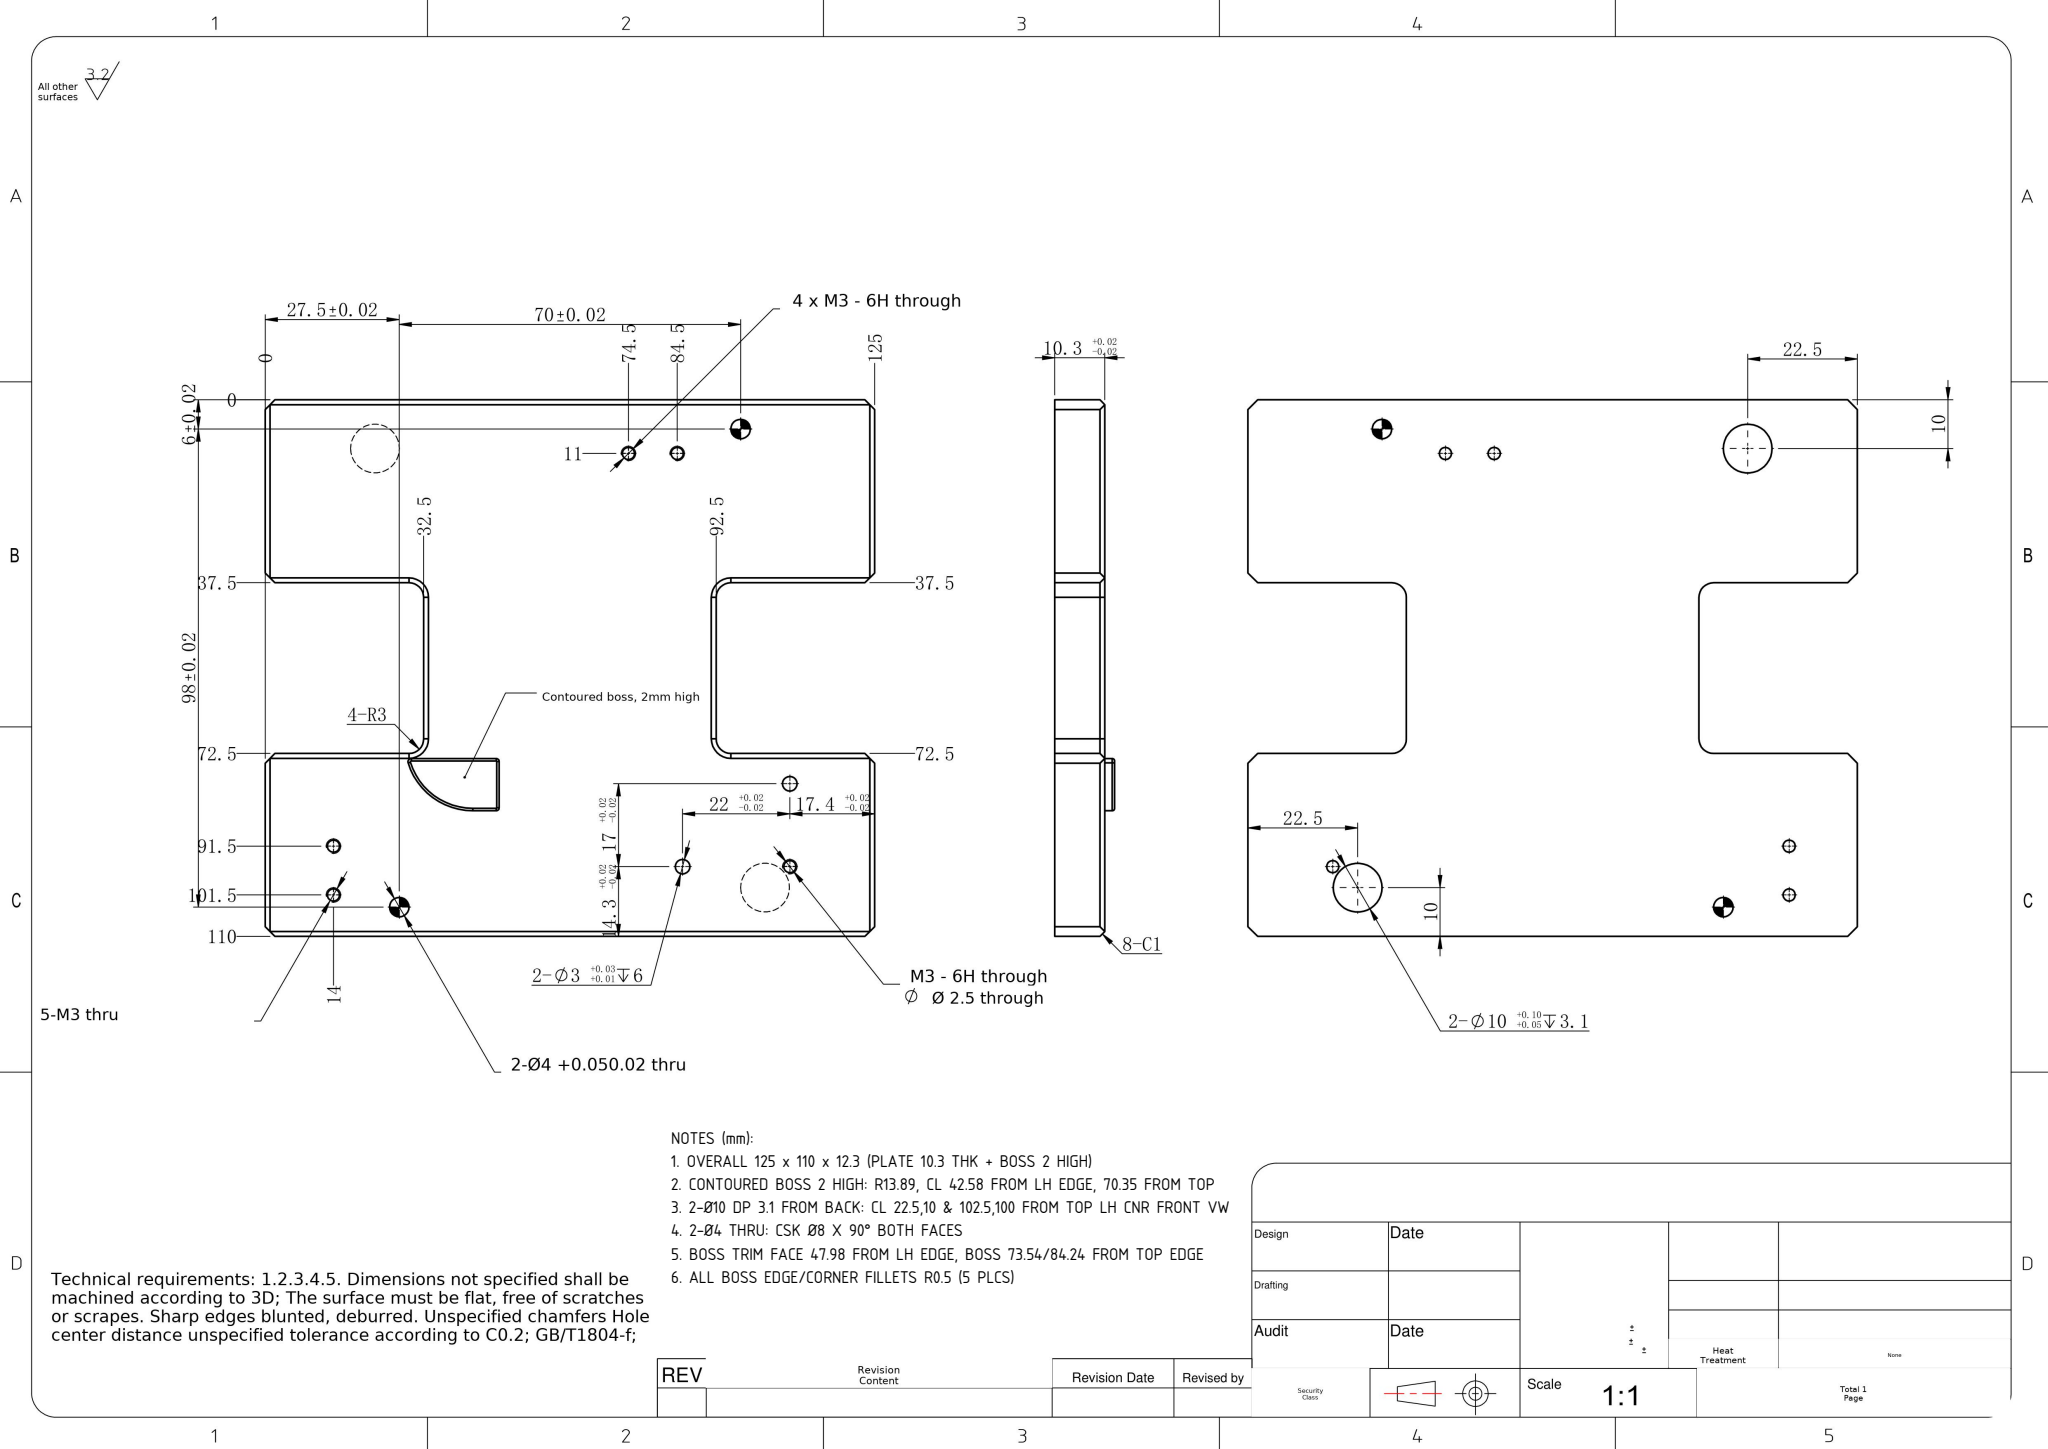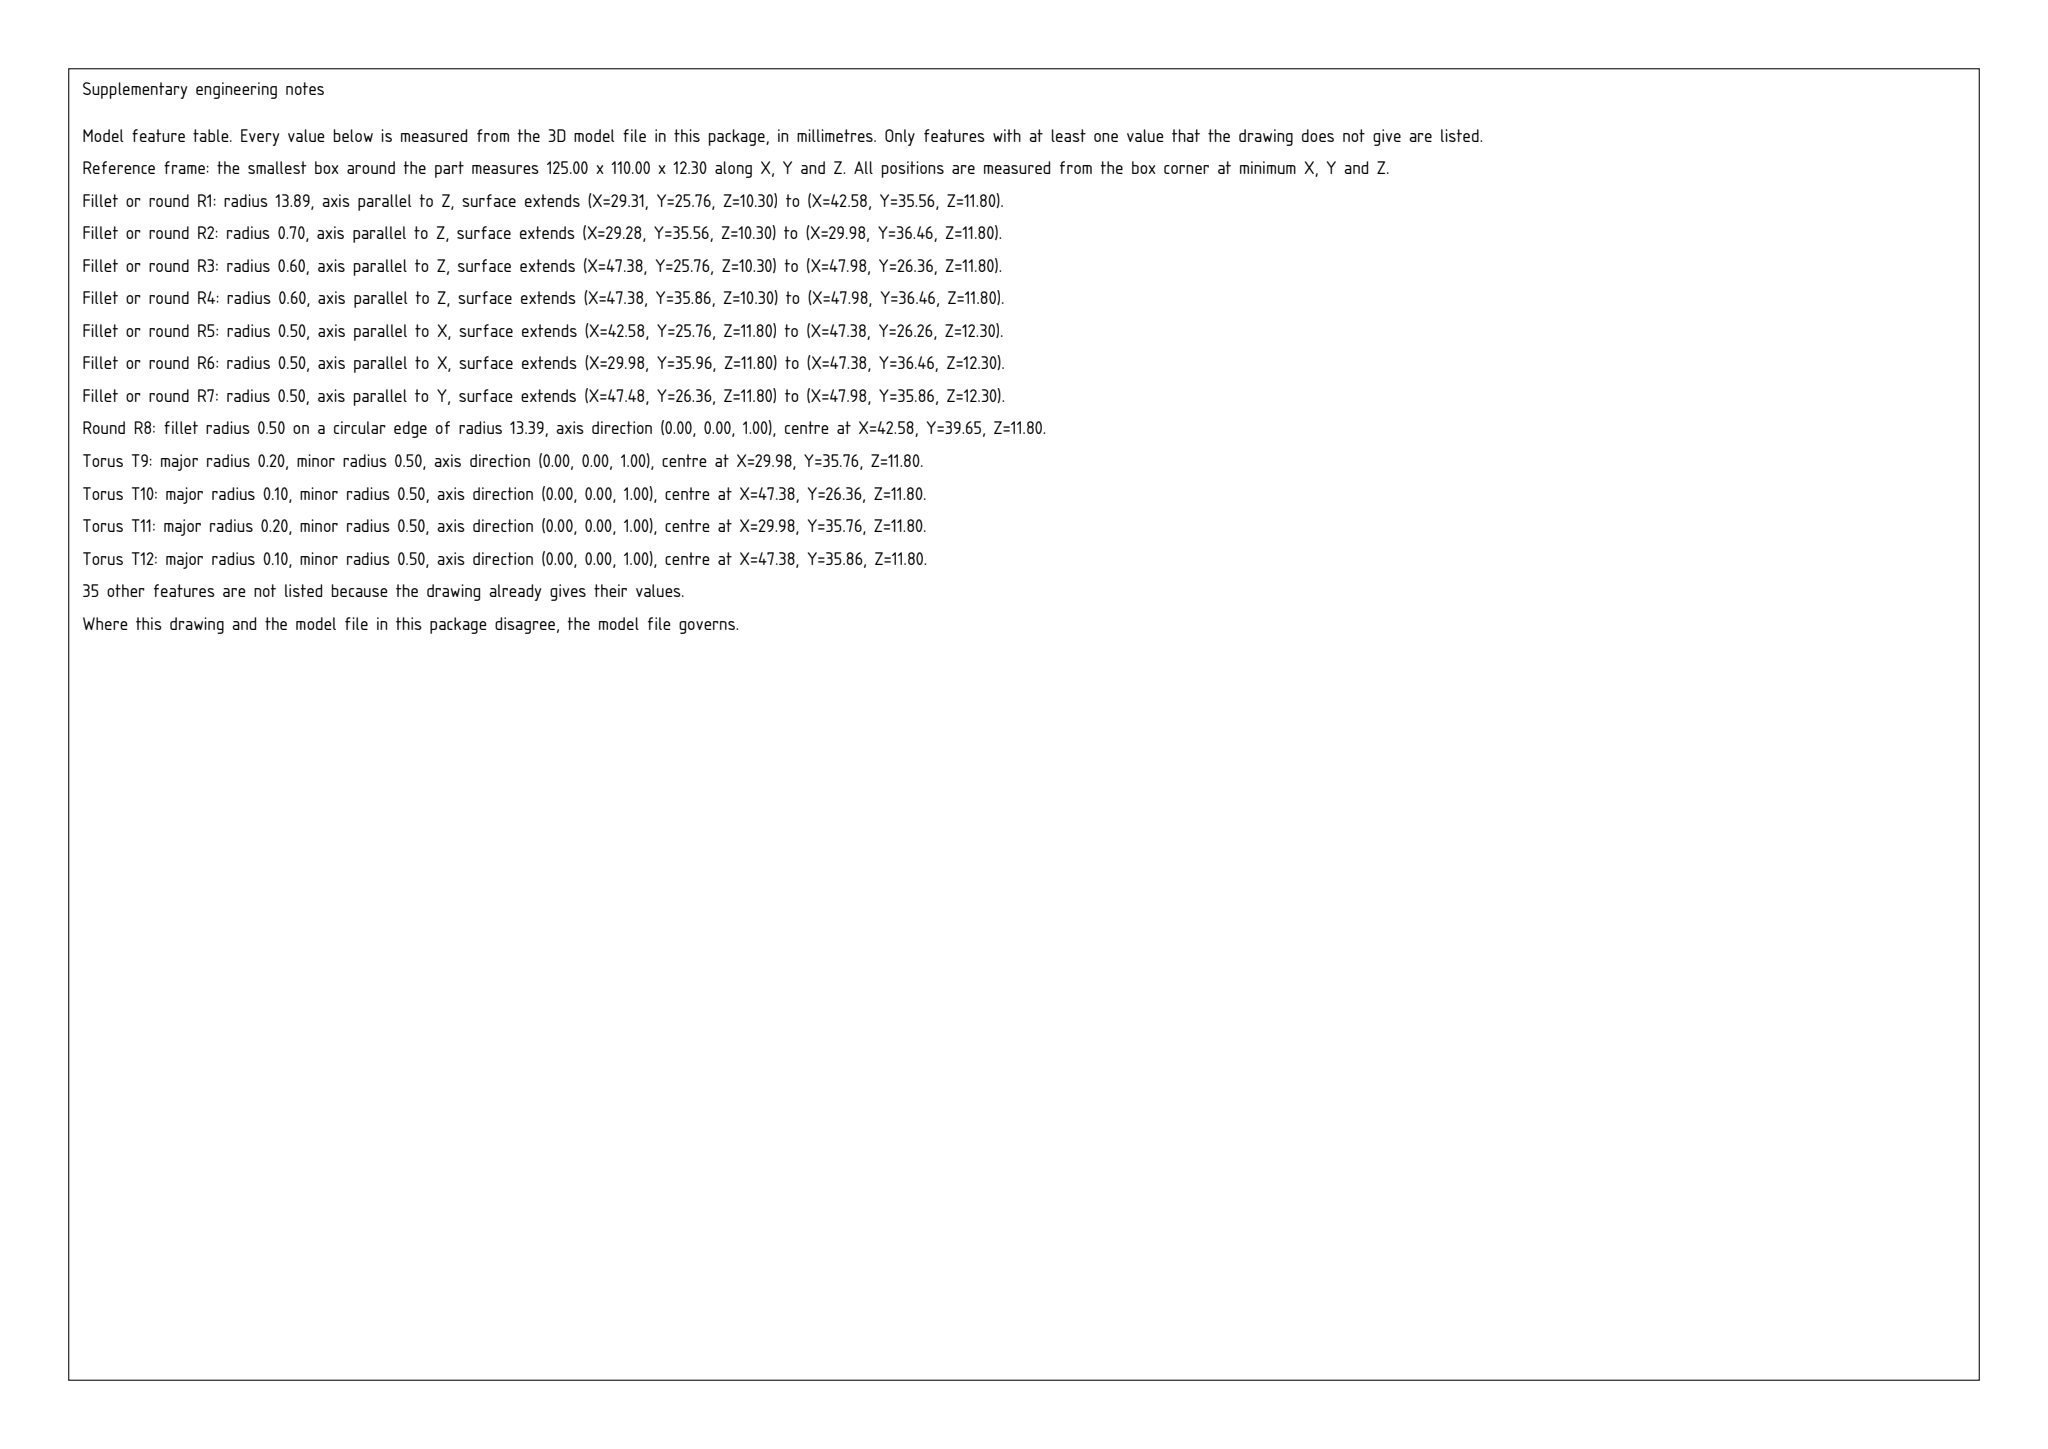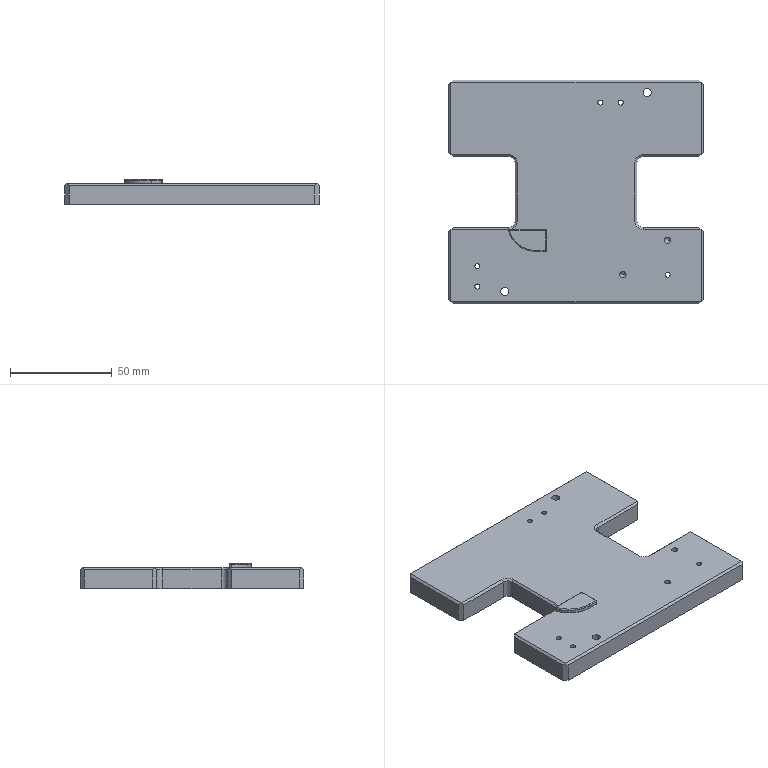Part | SolidWorks | mm | 1 solid | 87 faces | box 125 x 110 x 12.3 mm | volume 117062 mm3 | plane 40 | cylinder 34 | cone 8 | torus 5 | commonest cylinder face diameters 2.5 x10 10 x4 3 x4 4 x4 6 x4 1 x3 1.4 x2 1.2 x2
Drawing notes:
OVERALL 125 x 110 x 12.3 (PLATE 10.3 THK + BOSS 2 HIGH) | from the solid: bbox 125,110,12.3; z planes 0, 10.3, 12.3
CONTOURED BOSS 2 HIGH: R13.89, CL 42.58 FROM LH EDGE, 70.35 FROM TOP | from the solid: cyl dia 27.771 axis z at (42.58,39.65) len 1.5; z planes 10.3 & 12.3; 110-39.65=70.35
2-Ø10 DP 3.1 FROM BACK: CL 22.5,10 & 102.5,100 FROM TOP LH CNR FRONT VW | from the solid: cyl dia10 axis z at (22.5,100) & (102.5,10), len 3.1, z plane 3.1; 110-100=10, 110-10=100
2-Ø4 THRU: CSK Ø8 X 90° BOTH FACES | from the solid: cones [90.0,8.0] x4 on 4.0 dia z-holes at (27.5,6.0) and (97.5,104.0)
BOSS TRIM FACE 47.98 FROM LH EDGE, BOSS 73.54/84.24 FROM TOP EDGE | from the solid: axis_planes x=47.98; y=36.46 & y=25.76 (110-36.46=73.54, 110-25.76=84.24); boss arc Ø27.771 at x42.58, y39.65 (=70.35 from top)
ALL BOSS EDGE/CORNER FILLETS R0.5 (5 PLCS) | from the solid: fillet_radii [[0.5,5]]